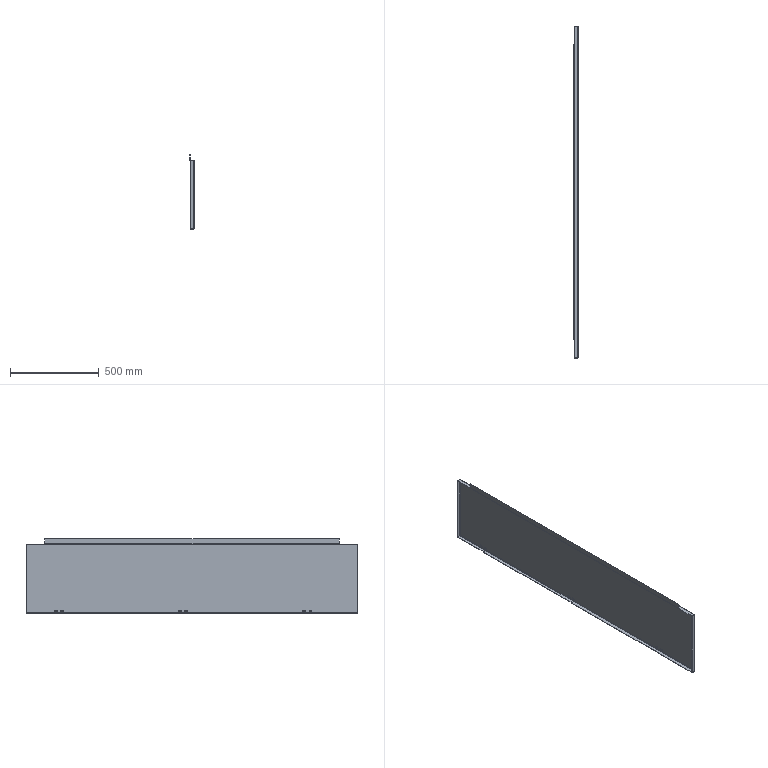Component | SolidWorks | RightFrontDoorAssembly-1_RightFrontDoorPanel06-03-1 | 1 solid | 86 faces | volume 1733971 mm3 | plane 44 | cylinder 34 | spline 8 | commonest cylinder face diameters 6 x24 5 x5 9 x5